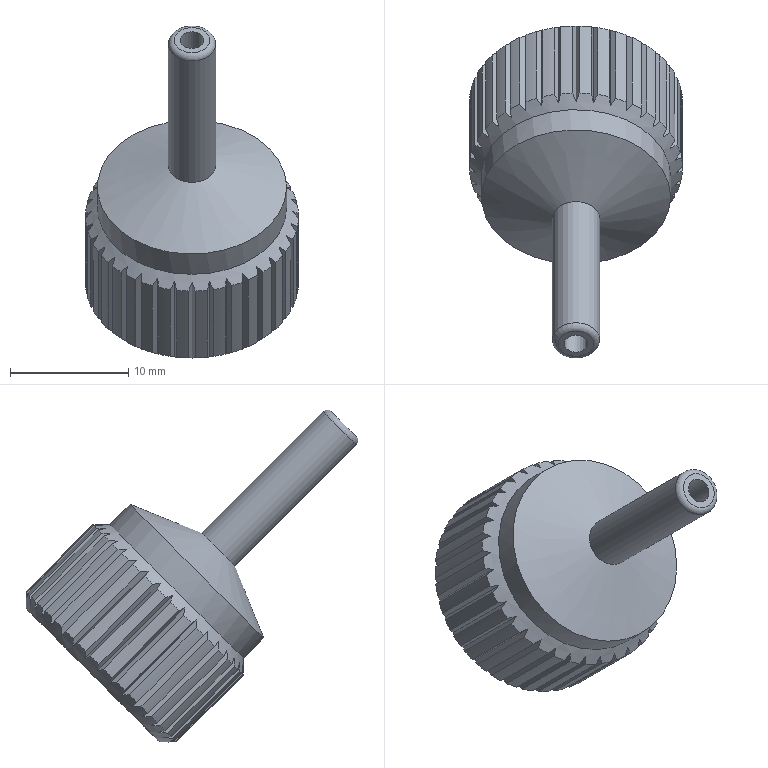Component | NX | NOZZLE | 1 solid | 130 faces | volume 2159 mm3 | plane 80 | cylinder 45 | cone 4 | torus 1 | commonest cylinder face diameters 18 x36 4 x1 10.75 x1 2 x1 16 x1 12 x1 14.04 x1 13.2 x1